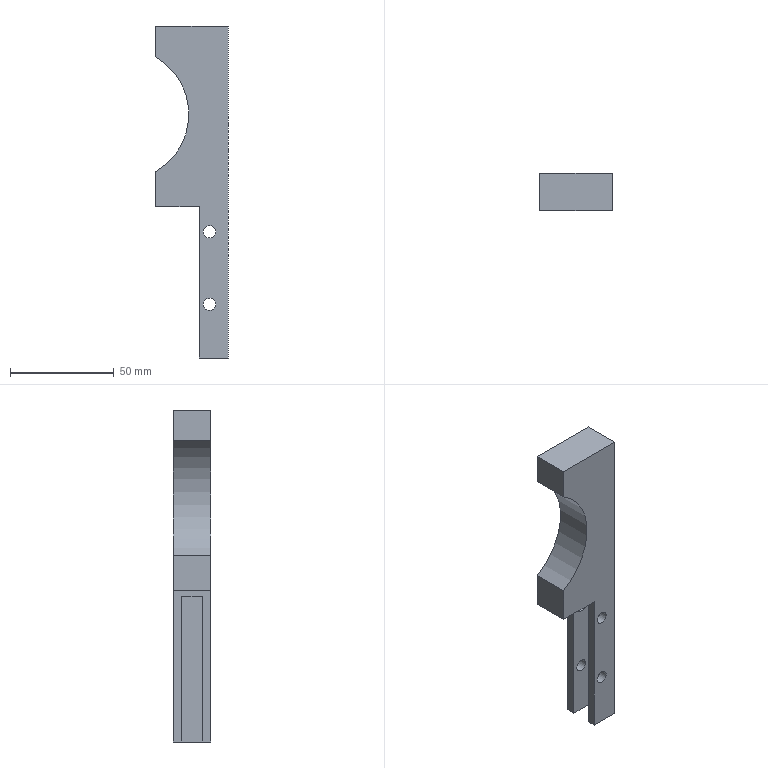Component | NX | JJZ-004 | 1 solid | 18 faces | volume 54508 mm3 | plane 13 | cylinder 5 | commonest cylinder face diameters 6 x4 64.071 x1